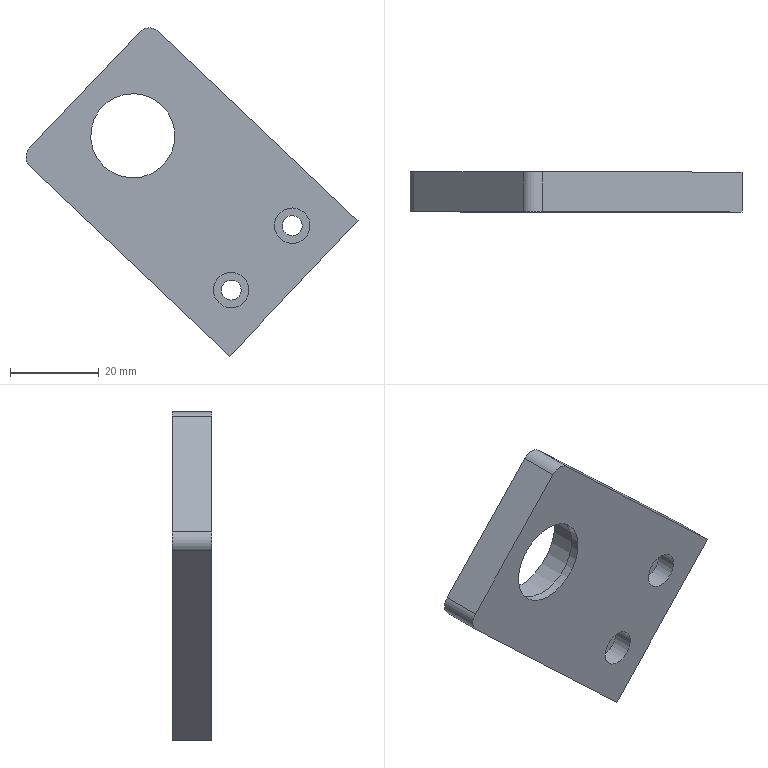Component | SolidWorks | 100-1_Copy(8)-1 | 1 solid | 23 faces | box 74.83 x 9 x 73.96 mm | volume 20712 mm3 | cylinder 14 | plane 9 | commonest cylinder face diameters 8 x4 4.5 x4 6 x2 22 x2 19 x2
STEP:
#1=CARTESIAN_POINT('',(18.66,42.205,-79.173));
#2=VERTEX_POINT('',#1);
#3=CARTESIAN_POINT('',(18.664,42.205,-79.34));
#4=VERTEX_POINT('',#3);
#5=CARTESIAN_POINT('',(18.746,42.205,-79.254));
#6=DIRECTION('',(0.,-1.,-0.));
#7=DIRECTION('',(-0.6879,0.,-0.7258));
#8=AXIS2_PLACEMENT_3D('',#5,#6,#7);
#9=CIRCLE('',#8,0.1181);
#10=EDGE_CURVE('',#2,#4,#9,.T.);
#11=ORIENTED_EDGE('',*,*,#10,.F.);
#12=CARTESIAN_POINT('',(18.66,42.559,-79.173));
#13=VERTEX_POINT('',#12);
#14=CARTESIAN_POINT('',(18.66,42.205,-79.173));
#15=DIRECTION('',(0.,-1.,-0.));
#16=VECTOR('',#15,39.37);
#17=LINE('',#14,#16);
#18=EDGE_CURVE('',#13,#2,#17,.T.);
#19=ORIENTED_EDGE('',*,*,#18,.F.);
#20=CARTESIAN_POINT('',(18.664,42.559,-79.34));
#21=VERTEX_POINT('',#20);
#22=CARTESIAN_POINT('',(18.746,42.559,-79.254));
#23=DIRECTION('',(-0.,1.,0.));
#24=DIRECTION('',(-0.6879,0.,-0.7258));
#25=AXIS2_PLACEMENT_3D('',#22,#23,#24);
#26=CIRCLE('',#25,0.1181);
#27=EDGE_CURVE('',#21,#13,#26,.T.);
#28=ORIENTED_EDGE('',*,*,#27,.F.);
#29=CARTESIAN_POINT('',(18.664,42.205,-79.34));
#30=DIRECTION('',(-0.,1.,0.));
#31=VECTOR('',#30,39.37);
#32=LINE('',#29,#31);
#33=EDGE_CURVE('',#4,#21,#32,.T.);
#34=ORIENTED_EDGE('',*,*,#33,.F.);
#35=EDGE_LOOP('',(#11,#19,#28,#34));
#36=FACE_OUTER_BOUND('',#35,.T.);
#37=CARTESIAN_POINT('',(18.746,42.205,-79.254));
#38=DIRECTION('',(-0.,1.,0.));
#39=DIRECTION('',(-0.6879,0.,-0.7258));
#40=AXIS2_PLACEMENT_3D('',#37,#38,#39);
#41=CYLINDRICAL_SURFACE('',#40,0.1181);
#42=ADVANCED_FACE('',(#36),#41,.T.);
#43=CARTESIAN_POINT('',(19.802,42.205,-78.14));
#44=VERTEX_POINT('',#43);
#45=CARTESIAN_POINT('',(19.635,42.205,-78.144));
#46=VERTEX_POINT('',#45);
#47=CARTESIAN_POINT('',(19.721,42.205,-78.226));
#48=DIRECTION('',(0.,-1.,-0.));
#49=DIRECTION('',(-0.6879,0.,-0.7258));
#50=AXIS2_PLACEMENT_3D('',#47,#48,#49);
#51=CIRCLE('',#50,0.1181);
#52=EDGE_CURVE('',#44,#46,#51,.T.);
#53=ORIENTED_EDGE('',*,*,#52,.F.);
#54=CARTESIAN_POINT('',(19.802,42.559,-78.14));
#55=VERTEX_POINT('',#54);
#56=CARTESIAN_POINT('',(19.802,42.205,-78.14));
#57=DIRECTION('',(0.,-1.,-0.));
#58=VECTOR('',#57,39.37);
#59=LINE('',#56,#58);
#60=EDGE_CURVE('',#55,#44,#59,.T.);
#61=ORIENTED_EDGE('',*,*,#60,.F.);
#62=CARTESIAN_POINT('',(19.635,42.559,-78.144));
#63=VERTEX_POINT('',#62);
#64=CARTESIAN_POINT('',(19.721,42.559,-78.226));
#65=DIRECTION('',(-0.,1.,0.));
#66=DIRECTION('',(-0.6879,0.,-0.7258));
#67=AXIS2_PLACEMENT_3D('',#64,#65,#66);
#68=CIRCLE('',#67,0.1181);
#69=EDGE_CURVE('',#63,#55,#68,.T.);
#70=ORIENTED_EDGE('',*,*,#69,.F.);
#71=CARTESIAN_POINT('',(19.635,42.205,-78.144));
#72=DIRECTION('',(-0.,1.,0.));
#73=VECTOR('',#72,39.37);
#74=LINE('',#71,#73);
#75=EDGE_CURVE('',#46,#63,#74,.T.);
#76=ORIENTED_EDGE('',*,*,#75,.F.);
#77=EDGE_LOOP('',(#53,#61,#70,#76));
#78=FACE_OUTER_BOUND('',#77,.T.);
#79=CARTESIAN_POINT('',(19.721,42.205,-78.226));
#80=DIRECTION('',(-0.,1.,0.));
#81=DIRECTION('',(-0.6879,0.,-0.7258));
#82=AXIS2_PLACEMENT_3D('',#79,#80,#81);
#83=CYLINDRICAL_SURFACE('',#82,0.1181);
#84=ADVANCED_FACE('',(#78),#83,.T.);
#85=CARTESIAN_POINT('',(19.319,42.283,-79.336));
#86=VERTEX_POINT('',#85);
#87=CARTESIAN_POINT('',(19.833,42.283,-78.793));
#88=VERTEX_POINT('',#87);
#89=CARTESIAN_POINT('',(19.576,42.283,-79.065));
#90=DIRECTION('',(-0.,1.,0.));
#91=DIRECTION('',(-0.6879,0.,-0.7258));
#92=AXIS2_PLACEMENT_3D('',#89,#90,#91);
#93=CIRCLE('',#92,0.374);
#94=EDGE_CURVE('',#86,#88,#93,.T.);
#95=ORIENTED_EDGE('',*,*,#94,.F.);
#96=CARTESIAN_POINT('',(19.576,42.283,-79.065));
#97=DIRECTION('',(-0.,1.,0.));
#98=DIRECTION('',(-0.6879,0.,-0.7258));
#99=AXIS2_PLACEMENT_3D('',#96,#97,#98);
#100=CIRCLE('',#99,0.374);
#101=EDGE_CURVE('',#88,#86,#100,.T.);
#102=ORIENTED_EDGE('',*,*,#101,.F.);
#103=EDGE_LOOP('',(#95,#102));
#104=FACE_BOUND('',#103,.T.);
#105=CARTESIAN_POINT('',(19.278,42.283,-79.379));
#106=VERTEX_POINT('',#105);
#107=CARTESIAN_POINT('',(19.874,42.283,-78.751));
#108=VERTEX_POINT('',#107);
#109=CARTESIAN_POINT('',(19.576,42.283,-79.065));
#110=DIRECTION('',(-0.,1.,0.));
#111=DIRECTION('',(-0.6879,0.,-0.7258));
#112=AXIS2_PLACEMENT_3D('',#109,#110,#111);
#113=CIRCLE('',#112,0.4331);
#114=EDGE_CURVE('',#106,#108,#113,.T.);
#115=ORIENTED_EDGE('',*,*,#114,.T.);
#116=CARTESIAN_POINT('',(19.576,42.283,-79.065));
#117=DIRECTION('',(-0.,1.,0.));
#118=DIRECTION('',(-0.6879,0.,-0.7258));
#119=AXIS2_PLACEMENT_3D('',#116,#117,#118);
#120=CIRCLE('',#119,0.4331);
#121=EDGE_CURVE('',#108,#106,#120,.T.);
#122=ORIENTED_EDGE('',*,*,#121,.T.);
#123=EDGE_LOOP('',(#115,#122));
#124=FACE_OUTER_BOUND('',#123,.T.);
#125=CARTESIAN_POINT('',(19.576,42.283,-79.065));
#126=DIRECTION('',(-0.,1.,0.));
#127=DIRECTION('',(0.7258,0.,-0.6879));
#128=AXIS2_PLACEMENT_3D('',#125,#126,#127);
#129=PLANE('',#128);
#130=ADVANCED_FACE('',(#104,#124),#129,.T.);
#131=CARTESIAN_POINT('',(19.874,42.559,-78.751));
#132=VERTEX_POINT('',#131);
#133=CARTESIAN_POINT('',(19.874,42.283,-78.751));
#134=DIRECTION('',(-0.,1.,0.));
#135=VECTOR('',#134,39.37);
#136=LINE('',#133,#135);
#137=EDGE_CURVE('',#108,#132,#136,.T.);
#138=ORIENTED_EDGE('',*,*,#137,.F.);
#139=ORIENTED_EDGE('',*,*,#114,.F.);
#140=CARTESIAN_POINT('',(19.278,42.559,-79.379));
#141=VERTEX_POINT('',#140);
#142=CARTESIAN_POINT('',(19.278,42.283,-79.379));
#143=DIRECTION('',(-0.,1.,0.));
#144=VECTOR('',#143,39.37);
#145=LINE('',#142,#144);
#146=EDGE_CURVE('',#106,#141,#145,.T.);
#147=ORIENTED_EDGE('',*,*,#146,.T.);
#148=CARTESIAN_POINT('',(19.576,42.559,-79.065));
#149=DIRECTION('',(-0.,1.,0.));
#150=DIRECTION('',(-0.6879,0.,-0.7258));
#151=AXIS2_PLACEMENT_3D('',#148,#149,#150);
#152=CIRCLE('',#151,0.4331);
#153=EDGE_CURVE('',#141,#132,#152,.T.);
#154=ORIENTED_EDGE('',*,*,#153,.T.);
#155=EDGE_LOOP('',(#138,#139,#147,#154));
#156=FACE_OUTER_BOUND('',#155,.T.);
#157=CARTESIAN_POINT('',(19.576,42.283,-79.065));
#158=DIRECTION('',(-0.,1.,0.));
#159=DIRECTION('',(-0.6879,0.,-0.7258));
#160=AXIS2_PLACEMENT_3D('',#157,#158,#159);
#161=CYLINDRICAL_SURFACE('',#160,0.4331);
#162=ADVANCED_FACE('',(#156),#161,.F.);
#163=CARTESIAN_POINT('',(20.34,42.382,-80.548));
#164=VERTEX_POINT('',#163);
#165=CARTESIAN_POINT('',(20.34,42.205,-80.548));
#166=VERTEX_POINT('',#165);
#167=CARTESIAN_POINT('',(20.34,42.205,-80.548));
#168=DIRECTION('',(0.,-1.,-0.));
#169=VECTOR('',#168,39.37);
#170=LINE('',#167,#169);
#171=EDGE_CURVE('',#164,#166,#170,.T.);
#172=ORIENTED_EDGE('',*,*,#171,.F.);
#173=CARTESIAN_POINT('',(20.557,42.382,-80.32));
#174=VERTEX_POINT('',#173);
#175=CARTESIAN_POINT('',(20.448,42.382,-80.434));
#176=DIRECTION('',(0.,-1.,-0.));
#177=DIRECTION('',(0.6879,0.,0.7258));
#178=AXIS2_PLACEMENT_3D('',#175,#176,#177);
#179=CIRCLE('',#178,0.1575);
#180=EDGE_CURVE('',#174,#164,#179,.T.);
#181=ORIENTED_EDGE('',*,*,#180,.F.);
#182=CARTESIAN_POINT('',(20.557,42.205,-80.32));
#183=VERTEX_POINT('',#182);
#184=CARTESIAN_POINT('',(20.557,42.205,-80.32));
#185=DIRECTION('',(0.,-1.,-0.));
#186=VECTOR('',#185,39.37);
#187=LINE('',#184,#186);
#188=EDGE_CURVE('',#174,#183,#187,.T.);
#189=ORIENTED_EDGE('',*,*,#188,.T.);
#190=CARTESIAN_POINT('',(20.448,42.205,-80.434));
#191=DIRECTION('',(0.,-1.,-0.));
#192=DIRECTION('',(0.6879,0.,0.7258));
#193=AXIS2_PLACEMENT_3D('',#190,#191,#192);
#194=CIRCLE('',#193,0.1575);
#195=EDGE_CURVE('',#183,#166,#194,.T.);
#196=ORIENTED_EDGE('',*,*,#195,.T.);
#197=EDGE_LOOP('',(#172,#181,#189,#196));
#198=FACE_OUTER_BOUND('',#197,.T.);
#199=CARTESIAN_POINT('',(20.448,42.205,-80.434));
#200=DIRECTION('',(0.,-1.,-0.));
#201=DIRECTION('',(0.6879,0.,0.7258));
#202=AXIS2_PLACEMENT_3D('',#199,#200,#201);
#203=CYLINDRICAL_SURFACE('',#202,0.1575);
#204=ADVANCED_FACE('',(#198),#203,.F.);
#205=CARTESIAN_POINT('',(20.509,42.382,-80.37));
#206=VERTEX_POINT('',#205);
#207=CARTESIAN_POINT('',(20.387,42.382,-80.498));
#208=VERTEX_POINT('',#207);
#209=CARTESIAN_POINT('',(20.448,42.382,-80.434));
#210=DIRECTION('',(0.,-1.,-0.));
#211=DIRECTION('',(0.6879,0.,0.7258));
#212=AXIS2_PLACEMENT_3D('',#209,#210,#211);
#213=CIRCLE('',#212,0.08858);
#214=EDGE_CURVE('',#206,#208,#213,.T.);
#215=ORIENTED_EDGE('',*,*,#214,.F.);
#216=CARTESIAN_POINT('',(20.448,42.382,-80.434));
#217=DIRECTION('',(0.,-1.,-0.));
#218=DIRECTION('',(0.6879,0.,0.7258));
#219=AXIS2_PLACEMENT_3D('',#216,#217,#218);
#220=CIRCLE('',#219,0.08858);
#221=EDGE_CURVE('',#208,#206,#220,.T.);
#222=ORIENTED_EDGE('',*,*,#221,.F.);
#223=EDGE_LOOP('',(#215,#222));
#224=FACE_BOUND('',#223,.T.);
#225=ORIENTED_EDGE('',*,*,#180,.T.);
#226=CARTESIAN_POINT('',(20.448,42.382,-80.434));
#227=DIRECTION('',(0.,-1.,-0.));
#228=DIRECTION('',(0.6879,0.,0.7258));
#229=AXIS2_PLACEMENT_3D('',#226,#227,#228);
#230=CIRCLE('',#229,0.1575);
#231=EDGE_CURVE('',#164,#174,#230,.T.);
#232=ORIENTED_EDGE('',*,*,#231,.T.);
#233=EDGE_LOOP('',(#225,#232));
#234=FACE_OUTER_BOUND('',#233,.T.);
#235=CARTESIAN_POINT('',(20.509,42.382,-80.37));
#236=DIRECTION('',(-0.,1.,0.));
#237=DIRECTION('',(0.7258,0.,-0.6879));
#238=AXIS2_PLACEMENT_3D('',#235,#236,#237);
#239=PLANE('',#238);
#240=ADVANCED_FACE('',(#224,#234),#239,.F.);
#241=CARTESIAN_POINT('',(20.387,42.559,-80.498));
#242=VERTEX_POINT('',#241);
#243=CARTESIAN_POINT('',(20.387,42.205,-80.498));
#244=DIRECTION('',(0.,-1.,-0.));
#245=VECTOR('',#244,39.37);
#246=LINE('',#243,#245);
#247=EDGE_CURVE('',#242,#208,#246,.T.);
#248=ORIENTED_EDGE('',*,*,#247,.F.);
#249=CARTESIAN_POINT('',(20.509,42.559,-80.37));
#250=VERTEX_POINT('',#249);
#251=CARTESIAN_POINT('',(20.448,42.559,-80.434));
#252=DIRECTION('',(0.,-1.,-0.));
#253=DIRECTION('',(0.6879,0.,0.7258));
#254=AXIS2_PLACEMENT_3D('',#251,#252,#253);
#255=CIRCLE('',#254,0.08858);
#256=EDGE_CURVE('',#250,#242,#255,.T.);
#257=ORIENTED_EDGE('',*,*,#256,.F.);
#258=CARTESIAN_POINT('',(20.509,42.205,-80.37));
#259=DIRECTION('',(0.,-1.,-0.));
#260=VECTOR('',#259,39.37);
#261=LINE('',#258,#260);
#262=EDGE_CURVE('',#250,#206,#261,.T.);
#263=ORIENTED_EDGE('',*,*,#262,.T.);
#264=ORIENTED_EDGE('',*,*,#214,.T.);
#265=EDGE_LOOP('',(#248,#257,#263,#264));
#266=FACE_OUTER_BOUND('',#265,.T.);
#267=CARTESIAN_POINT('',(20.448,42.205,-80.434));
#268=DIRECTION('',(0.,-1.,-0.));
#269=DIRECTION('',(0.6879,0.,0.7258));
#270=AXIS2_PLACEMENT_3D('',#267,#268,#269);
#271=CYLINDRICAL_SURFACE('',#270,0.08858);
#272=ADVANCED_FACE('',(#266),#271,.F.);
#273=CARTESIAN_POINT('',(20.882,42.382,-79.977));
#274=VERTEX_POINT('',#273);
#275=CARTESIAN_POINT('',(20.882,42.205,-79.977));
#276=VERTEX_POINT('',#275);
#277=CARTESIAN_POINT('',(20.882,42.205,-79.977));
#278=DIRECTION('',(0.,-1.,-0.));
#279=VECTOR('',#278,39.37);
#280=LINE('',#277,#279);
#281=EDGE_CURVE('',#274,#276,#280,.T.);
#282=ORIENTED_EDGE('',*,*,#281,.F.);
#283=CARTESIAN_POINT('',(21.098,42.382,-79.748));
#284=VERTEX_POINT('',#283);
#285=CARTESIAN_POINT('',(20.99,42.382,-79.862));
#286=DIRECTION('',(0.,-1.,-0.));
#287=DIRECTION('',(0.6879,0.,0.7258));
#288=AXIS2_PLACEMENT_3D('',#285,#286,#287);
#289=CIRCLE('',#288,0.1575);
#290=EDGE_CURVE('',#284,#274,#289,.T.);
#291=ORIENTED_EDGE('',*,*,#290,.F.);
#292=CARTESIAN_POINT('',(21.098,42.205,-79.748));
#293=VERTEX_POINT('',#292);
#294=CARTESIAN_POINT('',(21.098,42.205,-79.748));
#295=DIRECTION('',(0.,-1.,-0.));
#296=VECTOR('',#295,39.37);
#297=LINE('',#294,#296);
#298=EDGE_CURVE('',#284,#293,#297,.T.);
#299=ORIENTED_EDGE('',*,*,#298,.T.);
#300=CARTESIAN_POINT('',(20.99,42.205,-79.862));
#301=DIRECTION('',(0.,-1.,-0.));
#302=DIRECTION('',(0.6879,0.,0.7258));
#303=AXIS2_PLACEMENT_3D('',#300,#301,#302);
#304=CIRCLE('',#303,0.1575);
#305=EDGE_CURVE('',#293,#276,#304,.T.);
#306=ORIENTED_EDGE('',*,*,#305,.T.);
#307=EDGE_LOOP('',(#282,#291,#299,#306));
#308=FACE_OUTER_BOUND('',#307,.T.);
#309=CARTESIAN_POINT('',(20.99,42.205,-79.862));
#310=DIRECTION('',(0.,-1.,-0.));
#311=DIRECTION('',(0.6879,0.,0.7258));
#312=AXIS2_PLACEMENT_3D('',#309,#310,#311);
#313=CYLINDRICAL_SURFACE('',#312,0.1575);
#314=ADVANCED_FACE('',(#308),#313,.F.);
#315=CARTESIAN_POINT('',(21.051,42.382,-79.798));
#316=VERTEX_POINT('',#315);
#317=CARTESIAN_POINT('',(20.929,42.382,-79.927));
#318=VERTEX_POINT('',#317);
#319=CARTESIAN_POINT('',(20.99,42.382,-79.862));
#320=DIRECTION('',(0.,-1.,-0.));
#321=DIRECTION('',(0.6879,0.,0.7258));
#322=AXIS2_PLACEMENT_3D('',#319,#320,#321);
#323=CIRCLE('',#322,0.08858);
#324=EDGE_CURVE('',#316,#318,#323,.T.);
#325=ORIENTED_EDGE('',*,*,#324,.F.);
#326=CARTESIAN_POINT('',(20.99,42.382,-79.862));
#327=DIRECTION('',(0.,-1.,-0.));
#328=DIRECTION('',(0.6879,0.,0.7258));
#329=AXIS2_PLACEMENT_3D('',#326,#327,#328);
#330=CIRCLE('',#329,0.08858);
#331=EDGE_CURVE('',#318,#316,#330,.T.);
#332=ORIENTED_EDGE('',*,*,#331,.F.);
#333=EDGE_LOOP('',(#325,#332));
#334=FACE_BOUND('',#333,.T.);
#335=ORIENTED_EDGE('',*,*,#290,.T.);
#336=CARTESIAN_POINT('',(20.99,42.382,-79.862));
#337=DIRECTION('',(0.,-1.,-0.));
#338=DIRECTION('',(0.6879,0.,0.7258));
#339=AXIS2_PLACEMENT_3D('',#336,#337,#338);
#340=CIRCLE('',#339,0.1575);
#341=EDGE_CURVE('',#274,#284,#340,.T.);
#342=ORIENTED_EDGE('',*,*,#341,.T.);
#343=EDGE_LOOP('',(#335,#342));
#344=FACE_OUTER_BOUND('',#343,.T.);
#345=CARTESIAN_POINT('',(21.051,42.382,-79.798));
#346=DIRECTION('',(-0.,1.,0.));
#347=DIRECTION('',(0.7258,0.,-0.6879));
#348=AXIS2_PLACEMENT_3D('',#345,#346,#347);
#349=PLANE('',#348);
#350=ADVANCED_FACE('',(#334,#344),#349,.F.);
#351=CARTESIAN_POINT('',(20.929,42.559,-79.927));
#352=VERTEX_POINT('',#351);
#353=CARTESIAN_POINT('',(20.929,42.205,-79.927));
#354=DIRECTION('',(0.,-1.,-0.));
#355=VECTOR('',#354,39.37);
#356=LINE('',#353,#355);
#357=EDGE_CURVE('',#352,#318,#356,.T.);
#358=ORIENTED_EDGE('',*,*,#357,.F.);
#359=CARTESIAN_POINT('',(21.051,42.559,-79.798));
#360=VERTEX_POINT('',#359);
#361=CARTESIAN_POINT('',(20.99,42.559,-79.862));
#362=DIRECTION('',(0.,-1.,-0.));
#363=DIRECTION('',(0.6879,0.,0.7258));
#364=AXIS2_PLACEMENT_3D('',#361,#362,#363);
#365=CIRCLE('',#364,0.08858);
#366=EDGE_CURVE('',#360,#352,#365,.T.);
#367=ORIENTED_EDGE('',*,*,#366,.F.);
#368=CARTESIAN_POINT('',(21.051,42.205,-79.798));
#369=DIRECTION('',(0.,-1.,-0.));
#370=VECTOR('',#369,39.37);
#371=LINE('',#368,#370);
#372=EDGE_CURVE('',#360,#316,#371,.T.);
#373=ORIENTED_EDGE('',*,*,#372,.T.);
#374=ORIENTED_EDGE('',*,*,#324,.T.);
#375=EDGE_LOOP('',(#358,#367,#373,#374));
#376=FACE_OUTER_BOUND('',#375,.T.);
#377=CARTESIAN_POINT('',(20.99,42.205,-79.862));
#378=DIRECTION('',(0.,-1.,-0.));
#379=DIRECTION('',(0.6879,0.,0.7258));
#380=AXIS2_PLACEMENT_3D('',#377,#378,#379);
#381=CYLINDRICAL_SURFACE('',#380,0.08858);
#382=ADVANCED_FACE('',(#376),#381,.F.);
#383=CARTESIAN_POINT('',(20.436,42.559,-81.019));
#384=VERTEX_POINT('',#383);
#385=CARTESIAN_POINT('',(21.574,42.559,-79.819));
#386=VERTEX_POINT('',#385);
#387=CARTESIAN_POINT('',(20.436,42.559,-81.019));
#388=DIRECTION('',(0.6879,0.,0.7258));
#389=VECTOR('',#388,39.37);
#390=LINE('',#387,#389);
#391=EDGE_CURVE('',#384,#386,#390,.T.);
#392=ORIENTED_EDGE('',*,*,#391,.T.);
#393=CARTESIAN_POINT('',(21.574,42.205,-79.819));
#394=VERTEX_POINT('',#393);
#395=CARTESIAN_POINT('',(21.574,42.205,-79.819));
#396=DIRECTION('',(-0.,1.,0.));
#397=VECTOR('',#396,39.37);
#398=LINE('',#395,#397);
#399=EDGE_CURVE('',#394,#386,#398,.T.);
#400=ORIENTED_EDGE('',*,*,#399,.F.);
#401=CARTESIAN_POINT('',(20.436,42.205,-81.019));
#402=VERTEX_POINT('',#401);
#403=CARTESIAN_POINT('',(20.436,42.205,-81.019));
#404=DIRECTION('',(0.6879,0.,0.7258));
#405=VECTOR('',#404,39.37);
#406=LINE('',#403,#405);
#407=EDGE_CURVE('',#402,#394,#406,.T.);
#408=ORIENTED_EDGE('',*,*,#407,.F.);
#409=CARTESIAN_POINT('',(20.436,42.205,-81.019));
#410=DIRECTION('',(-0.,1.,0.));
#411=VECTOR('',#410,39.37);
#412=LINE('',#409,#411);
#413=EDGE_CURVE('',#402,#384,#412,.T.);
#414=ORIENTED_EDGE('',*,*,#413,.T.);
#415=EDGE_LOOP('',(#392,#400,#408,#414));
#416=FACE_OUTER_BOUND('',#415,.T.);
#417=CARTESIAN_POINT('',(20.436,42.205,-81.019));
#418=DIRECTION('',(-0.7258,-0.,0.6879));
#419=DIRECTION('',(0.6879,0.,0.7258));
#420=AXIS2_PLACEMENT_3D('',#417,#418,#419);
#421=PLANE('',#420);
#422=ADVANCED_FACE('',(#416),#421,.F.);
#423=CARTESIAN_POINT('',(20.436,42.205,-81.019));
#424=DIRECTION('',(0.7258,0.,-0.6879));
#425=VECTOR('',#424,39.37);
#426=LINE('',#423,#425);
#427=EDGE_CURVE('',#4,#402,#426,.T.);
#428=ORIENTED_EDGE('',*,*,#427,.F.);
#429=ORIENTED_EDGE('',*,*,#33,.T.);
#430=CARTESIAN_POINT('',(20.436,42.559,-81.019));
#431=DIRECTION('',(0.7258,0.,-0.6879));
#432=VECTOR('',#431,39.37);
#433=LINE('',#430,#432);
#434=EDGE_CURVE('',#21,#384,#433,.T.);
#435=ORIENTED_EDGE('',*,*,#434,.T.);
#436=ORIENTED_EDGE('',*,*,#413,.F.);
#437=EDGE_LOOP('',(#428,#429,#435,#436));
#438=FACE_OUTER_BOUND('',#437,.T.);
#439=CARTESIAN_POINT('',(20.436,42.205,-81.019));
#440=DIRECTION('',(0.6879,0.,0.7258));
#441=DIRECTION('',(0.7258,0.,-0.6879));
#442=AXIS2_PLACEMENT_3D('',#439,#440,#441);
#443=PLANE('',#442);
#444=ADVANCED_FACE('',(#438),#443,.F.);
#445=CARTESIAN_POINT('',(18.579,42.205,-79.259));
#446=DIRECTION('',(-0.6879,-0.,-0.7258));
#447=VECTOR('',#446,39.37);
#448=LINE('',#445,#447);
#449=EDGE_CURVE('',#46,#2,#448,.T.);
#450=ORIENTED_EDGE('',*,*,#449,.F.);
#451=ORIENTED_EDGE('',*,*,#75,.T.);
#452=CARTESIAN_POINT('',(18.579,42.559,-79.259));
#453=DIRECTION('',(-0.6879,-0.,-0.7258));
#454=VECTOR('',#453,39.37);
#455=LINE('',#452,#454);
#456=EDGE_CURVE('',#63,#13,#455,.T.);
#457=ORIENTED_EDGE('',*,*,#456,.T.);
#458=ORIENTED_EDGE('',*,*,#18,.T.);
#459=EDGE_LOOP('',(#450,#451,#457,#458));
#460=FACE_OUTER_BOUND('',#459,.T.);
#461=CARTESIAN_POINT('',(18.579,42.205,-79.259));
#462=DIRECTION('',(0.7258,0.,-0.6879));
#463=DIRECTION('',(-0.6879,-0.,-0.7258));
#464=AXIS2_PLACEMENT_3D('',#461,#462,#463);
#465=PLANE('',#464);
#466=ADVANCED_FACE('',(#460),#465,.F.);
#467=CARTESIAN_POINT('',(21.574,42.559,-79.819));
#468=DIRECTION('',(-0.7258,-0.,0.6879));
#469=VECTOR('',#468,39.37);
#470=LINE('',#467,#469);
#471=EDGE_CURVE('',#386,#55,#470,.T.);
#472=ORIENTED_EDGE('',*,*,#471,.T.);
#473=ORIENTED_EDGE('',*,*,#60,.T.);
#474=CARTESIAN_POINT('',(21.574,42.205,-79.819));
#475=DIRECTION('',(-0.7258,-0.,0.6879));
#476=VECTOR('',#475,39.37);
#477=LINE('',#474,#476);
#478=EDGE_CURVE('',#394,#44,#477,.T.);
#479=ORIENTED_EDGE('',*,*,#478,.F.);
#480=ORIENTED_EDGE('',*,*,#399,.T.);
#481=EDGE_LOOP('',(#472,#473,#479,#480));
#482=FACE_OUTER_BOUND('',#481,.T.);
#483=CARTESIAN_POINT('',(21.574,42.205,-79.819));
#484=DIRECTION('',(-0.6879,-0.,-0.7258));
#485=DIRECTION('',(-0.7258,-0.,0.6879));
#486=AXIS2_PLACEMENT_3D('',#483,#484,#485);
#487=PLANE('',#486);
#488=ADVANCED_FACE('',(#482),#487,.F.);
#489=ORIENTED_EDGE('',*,*,#366,.T.);
#490=CARTESIAN_POINT('',(20.99,42.559,-79.862));
#491=DIRECTION('',(0.,-1.,-0.));
#492=DIRECTION('',(0.6879,0.,0.7258));
#493=AXIS2_PLACEMENT_3D('',#490,#491,#492);
#494=CIRCLE('',#493,0.08858);
#495=EDGE_CURVE('',#352,#360,#494,.T.);
#496=ORIENTED_EDGE('',*,*,#495,.T.);
#497=EDGE_LOOP('',(#489,#496));
#498=FACE_BOUND('',#497,.T.);
#499=ORIENTED_EDGE('',*,*,#256,.T.);
#500=CARTESIAN_POINT('',(20.448,42.559,-80.434));
#501=DIRECTION('',(0.,-1.,-0.));
#502=DIRECTION('',(0.6879,0.,0.7258));
#503=AXIS2_PLACEMENT_3D('',#500,#501,#502);
#504=CIRCLE('',#503,0.08858);
#505=EDGE_CURVE('',#242,#250,#504,.T.);
#506=ORIENTED_EDGE('',*,*,#505,.T.);
#507=EDGE_LOOP('',(#499,#506));
#508=FACE_BOUND('',#507,.T.);
#509=ORIENTED_EDGE('',*,*,#153,.F.);
#510=CARTESIAN_POINT('',(19.576,42.559,-79.065));
#511=DIRECTION('',(-0.,1.,0.));
#512=DIRECTION('',(-0.6879,0.,-0.7258));
#513=AXIS2_PLACEMENT_3D('',#510,#511,#512);
#514=CIRCLE('',#513,0.4331);
#515=EDGE_CURVE('',#132,#141,#514,.T.);
#516=ORIENTED_EDGE('',*,*,#515,.F.);
#517=EDGE_LOOP('',(#509,#516));
#518=FACE_BOUND('',#517,.T.);
#519=ORIENTED_EDGE('',*,*,#456,.F.);
#520=ORIENTED_EDGE('',*,*,#69,.T.);
#521=ORIENTED_EDGE('',*,*,#471,.F.);
#522=ORIENTED_EDGE('',*,*,#391,.F.);
#523=ORIENTED_EDGE('',*,*,#434,.F.);
#524=ORIENTED_EDGE('',*,*,#27,.T.);
#525=EDGE_LOOP('',(#519,#520,#521,#522,#523,#524));
#526=FACE_OUTER_BOUND('',#525,.T.);
#527=CARTESIAN_POINT('',(20.076,42.559,-79.539));
#528=DIRECTION('',(-0.,1.,0.));
#529=DIRECTION('',(0.7258,0.,-0.6879));
#530=AXIS2_PLACEMENT_3D('',#527,#528,#529);
#531=PLANE('',#530);
#532=ADVANCED_FACE('',(#498,#508,#518,#526),#531,.T.);
#533=CARTESIAN_POINT('',(19.319,42.205,-79.336));
#534=VERTEX_POINT('',#533);
#535=CARTESIAN_POINT('',(19.833,42.205,-78.793));
#536=VERTEX_POINT('',#535);
#537=CARTESIAN_POINT('',(19.576,42.205,-79.065));
#538=DIRECTION('',(0.,-1.,-0.));
#539=DIRECTION('',(0.6879,0.,0.7258));
#540=AXIS2_PLACEMENT_3D('',#537,#538,#539);
#541=CIRCLE('',#540,0.374);
#542=EDGE_CURVE('',#534,#536,#541,.T.);
#543=ORIENTED_EDGE('',*,*,#542,.F.);
#544=CARTESIAN_POINT('',(19.576,42.205,-79.065));
#545=DIRECTION('',(0.,-1.,-0.));
#546=DIRECTION('',(0.6879,0.,0.7258));
#547=AXIS2_PLACEMENT_3D('',#544,#545,#546);
#548=CIRCLE('',#547,0.374);
#549=EDGE_CURVE('',#536,#534,#548,.T.);
#550=ORIENTED_EDGE('',*,*,#549,.F.);
#551=EDGE_LOOP('',(#543,#550));
#552=FACE_BOUND('',#551,.T.);
#553=ORIENTED_EDGE('',*,*,#305,.F.);
#554=CARTESIAN_POINT('',(20.99,42.205,-79.862));
#555=DIRECTION('',(0.,-1.,-0.));
#556=DIRECTION('',(0.6879,0.,0.7258));
#557=AXIS2_PLACEMENT_3D('',#554,#555,#556);
#558=CIRCLE('',#557,0.1575);
#559=EDGE_CURVE('',#276,#293,#558,.T.);
#560=ORIENTED_EDGE('',*,*,#559,.F.);
#561=EDGE_LOOP('',(#553,#560));
#562=FACE_BOUND('',#561,.T.);
#563=ORIENTED_EDGE('',*,*,#195,.F.);
#564=CARTESIAN_POINT('',(20.448,42.205,-80.434));
#565=DIRECTION('',(0.,-1.,-0.));
#566=DIRECTION('',(0.6879,0.,0.7258));
#567=AXIS2_PLACEMENT_3D('',#564,#565,#566);
#568=CIRCLE('',#567,0.1575);
#569=EDGE_CURVE('',#166,#183,#568,.T.);
#570=ORIENTED_EDGE('',*,*,#569,.F.);
#571=EDGE_LOOP('',(#563,#570));
#572=FACE_BOUND('',#571,.T.);
#573=ORIENTED_EDGE('',*,*,#478,.T.);
#574=ORIENTED_EDGE('',*,*,#52,.T.);
#575=ORIENTED_EDGE('',*,*,#449,.T.);
#576=ORIENTED_EDGE('',*,*,#10,.T.);
#577=ORIENTED_EDGE('',*,*,#427,.T.);
#578=ORIENTED_EDGE('',*,*,#407,.T.);
#579=EDGE_LOOP('',(#573,#574,#575,#576,#577,#578));
#580=FACE_OUTER_BOUND('',#579,.T.);
#581=CARTESIAN_POINT('',(20.076,42.205,-79.539));
#582=DIRECTION('',(-0.,1.,0.));
#583=DIRECTION('',(0.7258,0.,-0.6879));
#584=AXIS2_PLACEMENT_3D('',#581,#582,#583);
#585=PLANE('',#584);
#586=ADVANCED_FACE('',(#552,#562,#572,#580),#585,.F.);
#587=CARTESIAN_POINT('',(19.833,42.205,-78.793));
#588=DIRECTION('',(-0.,1.,0.));
#589=VECTOR('',#588,39.37);
#590=LINE('',#587,#589);
#591=EDGE_CURVE('',#536,#88,#590,.T.);
#592=ORIENTED_EDGE('',*,*,#591,.F.);
#593=ORIENTED_EDGE('',*,*,#549,.T.);
#594=CARTESIAN_POINT('',(19.319,42.205,-79.336));
#595=DIRECTION('',(-0.,1.,0.));
#596=VECTOR('',#595,39.37);
#597=LINE('',#594,#596);
#598=EDGE_CURVE('',#534,#86,#597,.T.);
#599=ORIENTED_EDGE('',*,*,#598,.T.);
#600=ORIENTED_EDGE('',*,*,#94,.T.);
#601=EDGE_LOOP('',(#592,#593,#599,#600));
#602=FACE_OUTER_BOUND('',#601,.T.);
#603=CARTESIAN_POINT('',(19.576,42.205,-79.065));
#604=DIRECTION('',(-0.,1.,0.));
#605=DIRECTION('',(-0.6879,0.,-0.7258));
#606=AXIS2_PLACEMENT_3D('',#603,#604,#605);
#607=CYLINDRICAL_SURFACE('',#606,0.374);
#608=ADVANCED_FACE('',(#602),#607,.F.);
#609=ORIENTED_EDGE('',*,*,#542,.T.);
#610=ORIENTED_EDGE('',*,*,#591,.T.);
#611=ORIENTED_EDGE('',*,*,#101,.T.);
#612=ORIENTED_EDGE('',*,*,#598,.F.);
#613=EDGE_LOOP('',(#609,#610,#611,#612));
#614=FACE_OUTER_BOUND('',#613,.T.);
#615=CARTESIAN_POINT('',(19.576,42.205,-79.065));
#616=DIRECTION('',(-0.,1.,0.));
#617=DIRECTION('',(-0.6879,0.,-0.7258));
#618=AXIS2_PLACEMENT_3D('',#615,#616,#617);
#619=CYLINDRICAL_SURFACE('',#618,0.374);
#620=ADVANCED_FACE('',(#614),#619,.F.);
#621=ORIENTED_EDGE('',*,*,#495,.F.);
#622=ORIENTED_EDGE('',*,*,#357,.T.);
#623=ORIENTED_EDGE('',*,*,#331,.T.);
#624=ORIENTED_EDGE('',*,*,#372,.F.);
#625=EDGE_LOOP('',(#621,#622,#623,#624));
#626=FACE_OUTER_BOUND('',#625,.T.);
#627=CARTESIAN_POINT('',(20.99,42.205,-79.862));
#628=DIRECTION('',(0.,-1.,-0.));
#629=DIRECTION('',(0.6879,0.,0.7258));
#630=AXIS2_PLACEMENT_3D('',#627,#628,#629);
#631=CYLINDRICAL_SURFACE('',#630,0.08858);
#632=ADVANCED_FACE('',(#626),#631,.F.);
#633=ORIENTED_EDGE('',*,*,#341,.F.);
#634=ORIENTED_EDGE('',*,*,#281,.T.);
#635=ORIENTED_EDGE('',*,*,#559,.T.);
#636=ORIENTED_EDGE('',*,*,#298,.F.);
#637=EDGE_LOOP('',(#633,#634,#635,#636));
#638=FACE_OUTER_BOUND('',#637,.T.);
#639=CARTESIAN_POINT('',(20.99,42.205,-79.862));
#640=DIRECTION('',(0.,-1.,-0.));
#641=DIRECTION('',(0.6879,0.,0.7258));
#642=AXIS2_PLACEMENT_3D('',#639,#640,#641);
#643=CYLINDRICAL_SURFACE('',#642,0.1575);
#644=ADVANCED_FACE('',(#638),#643,.F.);
#645=ORIENTED_EDGE('',*,*,#505,.F.);
#646=ORIENTED_EDGE('',*,*,#247,.T.);
#647=ORIENTED_EDGE('',*,*,#221,.T.);
#648=ORIENTED_EDGE('',*,*,#262,.F.);
#649=EDGE_LOOP('',(#645,#646,#647,#648));
#650=FACE_OUTER_BOUND('',#649,.T.);
#651=CARTESIAN_POINT('',(20.448,42.205,-80.434));
#652=DIRECTION('',(0.,-1.,-0.));
#653=DIRECTION('',(0.6879,0.,0.7258));
#654=AXIS2_PLACEMENT_3D('',#651,#652,#653);
#655=CYLINDRICAL_SURFACE('',#654,0.08858);
#656=ADVANCED_FACE('',(#650),#655,.F.);
#657=ORIENTED_EDGE('',*,*,#231,.F.);
#658=ORIENTED_EDGE('',*,*,#171,.T.);
#659=ORIENTED_EDGE('',*,*,#569,.T.);
#660=ORIENTED_EDGE('',*,*,#188,.F.);
#661=EDGE_LOOP('',(#657,#658,#659,#660));
#662=FACE_OUTER_BOUND('',#661,.T.);
#663=CARTESIAN_POINT('',(20.448,42.205,-80.434));
#664=DIRECTION('',(0.,-1.,-0.));
#665=DIRECTION('',(0.6879,0.,0.7258));
#666=AXIS2_PLACEMENT_3D('',#663,#664,#665);
#667=CYLINDRICAL_SURFACE('',#666,0.1575);
#668=ADVANCED_FACE('',(#662),#667,.F.);
#669=ORIENTED_EDGE('',*,*,#121,.F.);
#670=ORIENTED_EDGE('',*,*,#137,.T.);
#671=ORIENTED_EDGE('',*,*,#515,.T.);
#672=ORIENTED_EDGE('',*,*,#146,.F.);
#673=EDGE_LOOP('',(#669,#670,#671,#672));
#674=FACE_OUTER_BOUND('',#673,.T.);
#675=CARTESIAN_POINT('',(19.576,42.283,-79.065));
#676=DIRECTION('',(-0.,1.,0.));
#677=DIRECTION('',(-0.6879,0.,-0.7258));
#678=AXIS2_PLACEMENT_3D('',#675,#676,#677);
#679=CYLINDRICAL_SURFACE('',#678,0.4331);
#680=ADVANCED_FACE('',(#674),#679,.F.);
#681=CLOSED_SHELL('',(#42,#84,#130,#162,#204,#240,#272,#314,#350,#382,#422,#444,#466,#488,#532,#586,#608,#620,#632,#644,#656,#668,#680));
#682=MANIFOLD_SOLID_BREP('',#681);
#683=CARTESIAN_POINT('',(0.,0.,0.));
#684=DIRECTION('',(0.,0.,1.));
#685=DIRECTION('',(1.,0.,0.));
#686=AXIS2_PLACEMENT_3D('',#683,#684,#685);
#687=(LENGTH_UNIT()NAMED_UNIT(*)SI_UNIT($,.METRE.));
#688=LENGTH_MEASURE_WITH_UNIT(LENGTH_MEASURE(0.0254),#687);
#689=DIMENSIONAL_EXPONENTS(1.,0.,0.,0.,0.,0.,0.);
#690=(CONVERSION_BASED_UNIT('',#688)LENGTH_UNIT()NAMED_UNIT(#689));
#691=UNCERTAINTY_MEASURE_WITH_UNIT(LENGTH_MEASURE(0.00001),#690,'','');
#692=(NAMED_UNIT(*)PLANE_ANGLE_UNIT()SI_UNIT($,.RADIAN.));
#693=(NAMED_UNIT(*)SI_UNIT($,.STERADIAN.)SOLID_ANGLE_UNIT());
#694=(GEOMETRIC_REPRESENTATION_CONTEXT(3)GLOBAL_UNCERTAINTY_ASSIGNED_CONTEXT((#691))GLOBAL_UNIT_ASSIGNED_CONTEXT((#690,#692,#693))REPRESENTATION_CONTEXT('',''));
#695=ADVANCED_BREP_SHAPE_REPRESENTATION('',(#682,#686),#694);
#696=COLOUR_RGB('',0.7922,0.8196,0.9333);
#697=FILL_AREA_STYLE_COLOUR('',#696);
#698=FILL_AREA_STYLE('',(#697));
#699=SURFACE_STYLE_FILL_AREA(#698);
#700=SURFACE_SIDE_STYLE('',(#699));
#701=SURFACE_STYLE_USAGE(.BOTH.,#700);
#702=PRESENTATION_STYLE_ASSIGNMENT((#701));
#703=STYLED_ITEM('',(#702),#682);
#704=PRESENTATION_LAYER_ASSIGNMENT('','',(#703));
#705=(LENGTH_UNIT()NAMED_UNIT(*)SI_UNIT($,.METRE.));
#706=LENGTH_MEASURE_WITH_UNIT(LENGTH_MEASURE(0.0254),#705);
#707=DIMENSIONAL_EXPONENTS(1.,0.,0.,0.,0.,0.,0.);
#708=(CONVERSION_BASED_UNIT('',#706)LENGTH_UNIT()NAMED_UNIT(#707));
#709=UNCERTAINTY_MEASURE_WITH_UNIT(LENGTH_MEASURE(0.00001),#708,'','');
#710=(NAMED_UNIT(*)PLANE_ANGLE_UNIT()SI_UNIT($,.RADIAN.));
#711=(NAMED_UNIT(*)SI_UNIT($,.STERADIAN.)SOLID_ANGLE_UNIT());
#712=(GEOMETRIC_REPRESENTATION_CONTEXT(3)GLOBAL_UNCERTAINTY_ASSIGNED_CONTEXT((#709))GLOBAL_UNIT_ASSIGNED_CONTEXT((#708,#710,#711))REPRESENTATION_CONTEXT('',''));
#713=MECHANICAL_DESIGN_GEOMETRIC_PRESENTATION_REPRESENTATION('',(#703),#712);